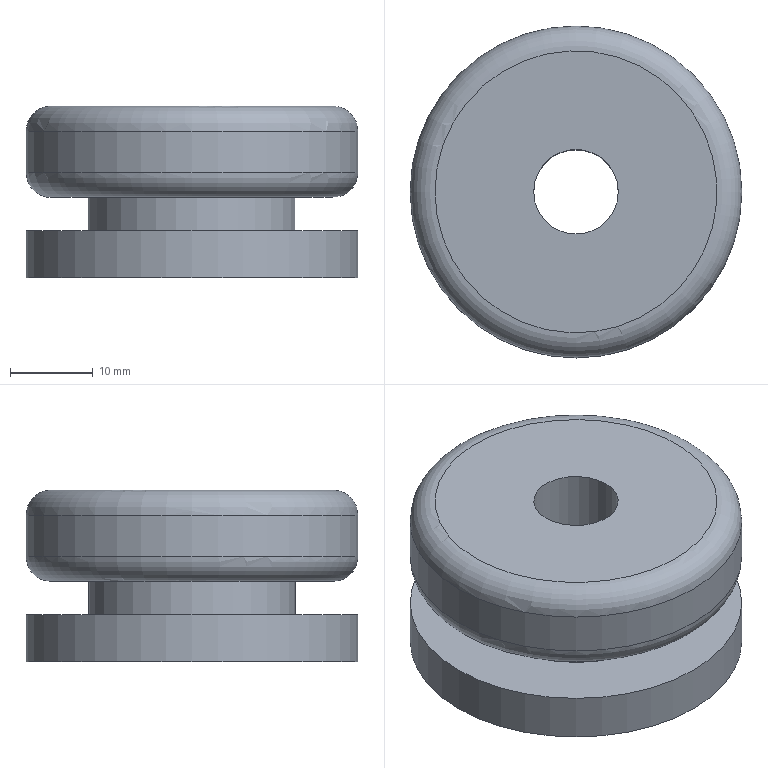Component | NX | RUBBER_PAD_3 | 1 solid | 10 faces | box 40 x 40 x 20.7 mm | volume 20789 mm3 | cylinder 4 | plane 4 | torus 2 | commonest cylinder face diameters 40 x2 10.2 x1 25 x1
STEP:
#1=CARTESIAN_POINT('',(0.,0.,0.));
#2=DIRECTION('',(0.,0.,1.));
#3=DIRECTION('',(1.,0.,0.));
#4=AXIS2_PLACEMENT_3D('',#1,#2,#3);
#5=CARTESIAN_POINT('',(-360.,342.5,-159.7));
#6=VERTEX_POINT('',#5);
#7=CARTESIAN_POINT('',(-340.,342.5,-159.7));
#8=DIRECTION('',(0.,0.,-1.));
#9=DIRECTION('',(-1.,0.,0.));
#10=AXIS2_PLACEMENT_3D('',#7,#8,#9);
#11=CIRCLE('',#10,20.);
#12=CARTESIAN_POINT('',(-340.,342.5,-150.));
#13=DIRECTION('',(0.,0.,-1.));
#14=DIRECTION('',(-1.,0.,0.));
#15=AXIS2_PLACEMENT_3D('',#12,#13,#14);
#16=CYLINDRICAL_SURFACE('',#15,20.);
#17=CARTESIAN_POINT('',(0.,9.7));
#18=DIRECTION('',(1.,0.));
#19=VECTOR('',#18,1.);
#20=LINE('',#17,#19);
#21=(GEOMETRIC_REPRESENTATION_CONTEXT(2)PARAMETRIC_REPRESENTATION_CONTEXT()REPRESENTATION_CONTEXT('',''));
#22=DEFINITIONAL_REPRESENTATION('',(#20),#21);
#23=PCURVE('',#16,#22);
#24=CARTESIAN_POINT('',(-340.,322.5,-159.7));
#25=DIRECTION('',(0.,0.,1.));
#26=DIRECTION('',(1.,0.,0.));
#27=AXIS2_PLACEMENT_3D('',#24,#25,#26);
#28=PLANE('',#27);
#29=CARTESIAN_POINT('',(-20.,20.));
#30=CARTESIAN_POINT('',(-20.,54.641));
#31=CARTESIAN_POINT('',(10.,37.321));
#32=CARTESIAN_POINT('',(40.,20.));
#33=CARTESIAN_POINT('',(10.,2.679));
#34=CARTESIAN_POINT('',(-20.,-14.641));
#35=CARTESIAN_POINT('',(-20.,20.));
#36=(BOUNDED_CURVE()B_SPLINE_CURVE(2,(#29,#30,#31,#32,#33,#34,#35),.UNSPECIFIED.,.T.,.F.)B_SPLINE_CURVE_WITH_KNOTS((1,2,2,2,2,1),(-2.094,0.,2.094,4.189,6.283,8.378),.UNSPECIFIED.)CURVE()GEOMETRIC_REPRESENTATION_ITEM()RATIONAL_B_SPLINE_CURVE((1.,0.5,1.,0.5,1.,0.5,1.))REPRESENTATION_ITEM(''));
#37=(GEOMETRIC_REPRESENTATION_CONTEXT(2)PARAMETRIC_REPRESENTATION_CONTEXT()REPRESENTATION_CONTEXT('',''));
#38=DEFINITIONAL_REPRESENTATION('',(#36),#37);
#39=PCURVE('',#28,#38);
#40=SURFACE_CURVE('',#11,(#23,#39),.PCURVE_S1.);
#41=EDGE_CURVE('',#6,#6,#40,.T.);
#42=ORIENTED_EDGE('',*,*,#41,.F.);
#43=CARTESIAN_POINT('',(-360.,342.5,-154.));
#44=VERTEX_POINT('',#43);
#45=CARTESIAN_POINT('',(-360.,342.5,-154.));
#46=CARTESIAN_POINT('',(-360.,342.5,-159.7));
#47=B_SPLINE_CURVE_WITH_KNOTS('',1,(#45,#46),.UNSPECIFIED.,.F.,.F.,(2,2),(4.,9.7),.PIECEWISE_BEZIER_KNOTS.);
#48=CARTESIAN_POINT('',(0.,0.));
#49=DIRECTION('',(0.,1.));
#50=VECTOR('',#49,1.);
#51=LINE('',#48,#50);
#52=(GEOMETRIC_REPRESENTATION_CONTEXT(2)PARAMETRIC_REPRESENTATION_CONTEXT()REPRESENTATION_CONTEXT('',''));
#53=DEFINITIONAL_REPRESENTATION('',(#51),#52);
#54=PCURVE('',#16,#53);
#55=CARTESIAN_POINT('',(6.283,0.));
#56=DIRECTION('',(0.,1.));
#57=VECTOR('',#56,1.);
#58=LINE('',#55,#57);
#59=(GEOMETRIC_REPRESENTATION_CONTEXT(2)PARAMETRIC_REPRESENTATION_CONTEXT()REPRESENTATION_CONTEXT('',''));
#60=DEFINITIONAL_REPRESENTATION('',(#58),#59);
#61=PCURVE('',#16,#60);
#62=SEAM_CURVE('',#47,(#54,#61),.PCURVE_S1.);
#63=EDGE_CURVE('',#44,#6,#62,.T.);
#64=ORIENTED_EDGE('',*,*,#63,.F.);
#65=CARTESIAN_POINT('',(-340.,342.5,-154.));
#66=DIRECTION('',(0.,0.,-1.));
#67=DIRECTION('',(-1.,0.,0.));
#68=AXIS2_PLACEMENT_3D('',#65,#66,#67);
#69=CIRCLE('',#68,20.);
#70=CARTESIAN_POINT('',(0.,4.));
#71=DIRECTION('',(1.,0.));
#72=VECTOR('',#71,1.);
#73=LINE('',#70,#72);
#74=(GEOMETRIC_REPRESENTATION_CONTEXT(2)PARAMETRIC_REPRESENTATION_CONTEXT()REPRESENTATION_CONTEXT('',''));
#75=DEFINITIONAL_REPRESENTATION('',(#73),#74);
#76=PCURVE('',#16,#75);
#77=CARTESIAN_POINT('',(-340.,330.,-154.));
#78=DIRECTION('',(0.,0.,-1.));
#79=DIRECTION('',(-1.,0.,0.));
#80=AXIS2_PLACEMENT_3D('',#77,#78,#79);
#81=PLANE('',#80);
#82=CARTESIAN_POINT('',(0.,12.5));
#83=DIRECTION('',(1.,0.));
#84=AXIS2_PLACEMENT_2D('',#82,#83);
#85=CIRCLE('',#84,20.);
#86=(GEOMETRIC_REPRESENTATION_CONTEXT(2)PARAMETRIC_REPRESENTATION_CONTEXT()REPRESENTATION_CONTEXT('',''));
#87=DEFINITIONAL_REPRESENTATION('',(#85),#86);
#88=PCURVE('',#81,#87);
#89=SURFACE_CURVE('',#69,(#76,#88),.PCURVE_S1.);
#90=EDGE_CURVE('',#44,#44,#89,.T.);
#91=ORIENTED_EDGE('',*,*,#90,.T.);
#92=ORIENTED_EDGE('',*,*,#63,.T.);
#93=EDGE_LOOP('',(#42,#64,#91,#92));
#94=FACE_BOUND('',#93,.T.);
#95=ADVANCED_FACE('',(#94),#16,.T.);
#96=CARTESIAN_POINT('',(-345.1,342.5,-159.7));
#97=VERTEX_POINT('',#96);
#98=CARTESIAN_POINT('',(-340.,342.5,-159.7));
#99=DIRECTION('',(0.,0.,-1.));
#100=DIRECTION('',(-1.,0.,0.));
#101=AXIS2_PLACEMENT_3D('',#98,#99,#100);
#102=CIRCLE('',#101,5.1);
#103=CARTESIAN_POINT('',(-5.1,20.));
#104=CARTESIAN_POINT('',(-5.1,28.833));
#105=CARTESIAN_POINT('',(2.55,24.417));
#106=CARTESIAN_POINT('',(10.2,20.));
#107=CARTESIAN_POINT('',(2.55,15.583));
#108=CARTESIAN_POINT('',(-5.1,11.167));
#109=CARTESIAN_POINT('',(-5.1,20.));
#110=(BOUNDED_CURVE()B_SPLINE_CURVE(2,(#103,#104,#105,#106,#107,#108,#109),.UNSPECIFIED.,.T.,.F.)B_SPLINE_CURVE_WITH_KNOTS((1,2,2,2,2,1),(-2.094,0.,2.094,4.189,6.283,8.378),.UNSPECIFIED.)CURVE()GEOMETRIC_REPRESENTATION_ITEM()RATIONAL_B_SPLINE_CURVE((1.,0.5,1.,0.5,1.,0.5,1.))REPRESENTATION_ITEM(''));
#111=(GEOMETRIC_REPRESENTATION_CONTEXT(2)PARAMETRIC_REPRESENTATION_CONTEXT()REPRESENTATION_CONTEXT('',''));
#112=DEFINITIONAL_REPRESENTATION('',(#110),#111);
#113=PCURVE('',#28,#112);
#114=CARTESIAN_POINT('',(-340.,342.5,-150.));
#115=DIRECTION('',(0.,0.,-1.));
#116=DIRECTION('',(-1.,0.,0.));
#117=AXIS2_PLACEMENT_3D('',#114,#115,#116);
#118=CYLINDRICAL_SURFACE('',#117,5.1);
#119=CARTESIAN_POINT('',(0.,9.7));
#120=DIRECTION('',(1.,0.));
#121=VECTOR('',#120,1.);
#122=LINE('',#119,#121);
#123=(GEOMETRIC_REPRESENTATION_CONTEXT(2)PARAMETRIC_REPRESENTATION_CONTEXT()REPRESENTATION_CONTEXT('',''));
#124=DEFINITIONAL_REPRESENTATION('',(#122),#123);
#125=PCURVE('',#118,#124);
#126=SURFACE_CURVE('',#102,(#113,#125),.PCURVE_S1.);
#127=EDGE_CURVE('',#97,#97,#126,.T.);
#128=ORIENTED_EDGE('',*,*,#127,.F.);
#129=EDGE_LOOP('',(#128));
#130=FACE_BOUND('',#129,.T.);
#131=ORIENTED_EDGE('',*,*,#41,.T.);
#132=EDGE_LOOP('',(#131));
#133=FACE_BOUND('',#132,.T.);
#134=ADVANCED_FACE('',(#130,#133),#28,.F.);
#135=CARTESIAN_POINT('',(-345.1,342.5,-139.));
#136=VERTEX_POINT('',#135);
#137=CARTESIAN_POINT('',(-340.,342.5,-139.));
#138=DIRECTION('',(0.,0.,-1.));
#139=DIRECTION('',(-1.,0.,0.));
#140=AXIS2_PLACEMENT_3D('',#137,#138,#139);
#141=CIRCLE('',#140,5.1);
#142=CARTESIAN_POINT('',(0.,-11.));
#143=DIRECTION('',(1.,0.));
#144=VECTOR('',#143,1.);
#145=LINE('',#142,#144);
#146=(GEOMETRIC_REPRESENTATION_CONTEXT(2)PARAMETRIC_REPRESENTATION_CONTEXT()REPRESENTATION_CONTEXT('',''));
#147=DEFINITIONAL_REPRESENTATION('',(#145),#146);
#148=PCURVE('',#118,#147);
#149=CARTESIAN_POINT('',(-340.,337.4,-139.));
#150=DIRECTION('',(0.,0.,-1.));
#151=DIRECTION('',(-1.,0.,0.));
#152=AXIS2_PLACEMENT_3D('',#149,#150,#151);
#153=PLANE('',#152);
#154=CARTESIAN_POINT('',(0.,5.1));
#155=DIRECTION('',(1.,0.));
#156=AXIS2_PLACEMENT_2D('',#154,#155);
#157=CIRCLE('',#156,5.1);
#158=(GEOMETRIC_REPRESENTATION_CONTEXT(2)PARAMETRIC_REPRESENTATION_CONTEXT()REPRESENTATION_CONTEXT('',''));
#159=DEFINITIONAL_REPRESENTATION('',(#157),#158);
#160=PCURVE('',#153,#159);
#161=SURFACE_CURVE('',#141,(#148,#160),.PCURVE_S1.);
#162=EDGE_CURVE('',#136,#136,#161,.T.);
#163=ORIENTED_EDGE('',*,*,#162,.T.);
#164=CARTESIAN_POINT('',(-345.1,342.5,-139.));
#165=CARTESIAN_POINT('',(-345.1,342.5,-159.7));
#166=B_SPLINE_CURVE_WITH_KNOTS('',1,(#164,#165),.UNSPECIFIED.,.F.,.F.,(2,2),(-11.,9.7),.PIECEWISE_BEZIER_KNOTS.);
#167=CARTESIAN_POINT('',(6.283,0.));
#168=DIRECTION('',(0.,1.));
#169=VECTOR('',#168,1.);
#170=LINE('',#167,#169);
#171=(GEOMETRIC_REPRESENTATION_CONTEXT(2)PARAMETRIC_REPRESENTATION_CONTEXT()REPRESENTATION_CONTEXT('',''));
#172=DEFINITIONAL_REPRESENTATION('',(#170),#171);
#173=PCURVE('',#118,#172);
#174=CARTESIAN_POINT('',(0.,0.));
#175=DIRECTION('',(0.,1.));
#176=VECTOR('',#175,1.);
#177=LINE('',#174,#176);
#178=(GEOMETRIC_REPRESENTATION_CONTEXT(2)PARAMETRIC_REPRESENTATION_CONTEXT()REPRESENTATION_CONTEXT('',''));
#179=DEFINITIONAL_REPRESENTATION('',(#177),#178);
#180=PCURVE('',#118,#179);
#181=SEAM_CURVE('',#166,(#173,#180),.PCURVE_S1.);
#182=EDGE_CURVE('',#136,#97,#181,.T.);
#183=ORIENTED_EDGE('',*,*,#182,.T.);
#184=ORIENTED_EDGE('',*,*,#127,.F.);
#185=ORIENTED_EDGE('',*,*,#182,.F.);
#186=EDGE_LOOP('',(#163,#183,#184,#185));
#187=FACE_BOUND('',#186,.F.);
#188=ADVANCED_FACE('',(#187),#118,.F.);
#189=CARTESIAN_POINT('',(-357.,342.5,-139.));
#190=VERTEX_POINT('',#189);
#191=CARTESIAN_POINT('',(-340.,342.5,-139.));
#192=DIRECTION('',(0.,0.,-1.));
#193=DIRECTION('',(-1.,0.,0.));
#194=AXIS2_PLACEMENT_3D('',#191,#192,#193);
#195=CIRCLE('',#194,17.);
#196=CARTESIAN_POINT('',(0.,5.1));
#197=DIRECTION('',(1.,0.));
#198=AXIS2_PLACEMENT_2D('',#196,#197);
#199=CIRCLE('',#198,17.);
#200=(GEOMETRIC_REPRESENTATION_CONTEXT(2)PARAMETRIC_REPRESENTATION_CONTEXT()REPRESENTATION_CONTEXT('',''));
#201=DEFINITIONAL_REPRESENTATION('',(#199),#200);
#202=PCURVE('',#153,#201);
#203=CARTESIAN_POINT('',(-340.,342.5,-142.));
#204=DIRECTION('',(0.,0.,-1.));
#205=DIRECTION('',(-1.,0.,0.));
#206=AXIS2_PLACEMENT_3D('',#203,#204,#205);
#207=TOROIDAL_SURFACE('',#206,17.,3.);
#208=CARTESIAN_POINT('',(0.,4.712));
#209=DIRECTION('',(1.,0.));
#210=VECTOR('',#209,1.);
#211=LINE('',#208,#210);
#212=(GEOMETRIC_REPRESENTATION_CONTEXT(2)PARAMETRIC_REPRESENTATION_CONTEXT()REPRESENTATION_CONTEXT('',''));
#213=DEFINITIONAL_REPRESENTATION('',(#211),#212);
#214=PCURVE('',#207,#213);
#215=SURFACE_CURVE('',#195,(#202,#214),.PCURVE_S1.);
#216=EDGE_CURVE('',#190,#190,#215,.T.);
#217=ORIENTED_EDGE('',*,*,#216,.F.);
#218=EDGE_LOOP('',(#217));
#219=FACE_BOUND('',#218,.T.);
#220=ORIENTED_EDGE('',*,*,#162,.T.);
#221=EDGE_LOOP('',(#220));
#222=FACE_BOUND('',#221,.T.);
#223=ADVANCED_FACE('',(#219,#222),#153,.F.);
#224=CARTESIAN_POINT('',(-360.,342.5,-142.));
#225=VERTEX_POINT('',#224);
#226=CARTESIAN_POINT('',(-340.,342.5,-142.));
#227=DIRECTION('',(0.,0.,-1.));
#228=DIRECTION('',(-1.,0.,0.));
#229=AXIS2_PLACEMENT_3D('',#226,#227,#228);
#230=CIRCLE('',#229,20.);
#231=CARTESIAN_POINT('',(0.,6.283));
#232=DIRECTION('',(1.,0.));
#233=VECTOR('',#232,1.);
#234=LINE('',#231,#233);
#235=(GEOMETRIC_REPRESENTATION_CONTEXT(2)PARAMETRIC_REPRESENTATION_CONTEXT()REPRESENTATION_CONTEXT('',''));
#236=DEFINITIONAL_REPRESENTATION('',(#234),#235);
#237=PCURVE('',#207,#236);
#238=CARTESIAN_POINT('',(-340.,342.5,-150.));
#239=DIRECTION('',(0.,0.,-1.));
#240=DIRECTION('',(-1.,0.,0.));
#241=AXIS2_PLACEMENT_3D('',#238,#239,#240);
#242=CYLINDRICAL_SURFACE('',#241,20.);
#243=CARTESIAN_POINT('',(0.,-8.));
#244=DIRECTION('',(1.,0.));
#245=VECTOR('',#244,1.);
#246=LINE('',#243,#245);
#247=(GEOMETRIC_REPRESENTATION_CONTEXT(2)PARAMETRIC_REPRESENTATION_CONTEXT()REPRESENTATION_CONTEXT('',''));
#248=DEFINITIONAL_REPRESENTATION('',(#246),#247);
#249=PCURVE('',#242,#248);
#250=SURFACE_CURVE('',#230,(#237,#249),.PCURVE_S1.);
#251=EDGE_CURVE('',#225,#225,#250,.T.);
#252=ORIENTED_EDGE('',*,*,#251,.F.);
#253=CARTESIAN_POINT('',(-357.,342.5,-139.));
#254=CARTESIAN_POINT('',(-357.802,342.5,-139.));
#255=CARTESIAN_POINT('',(-358.583,342.5,-139.255));
#256=CARTESIAN_POINT('',(-359.256,342.5,-139.744));
#257=CARTESIAN_POINT('',(-359.745,342.5,-140.417));
#258=CARTESIAN_POINT('',(-360.,342.5,-141.198));
#259=CARTESIAN_POINT('',(-360.,342.5,-142.));
#260=(BOUNDED_CURVE()B_SPLINE_CURVE(6,(#253,#254,#255,#256,#257,#258,#259),.UNSPECIFIED.,.F.,.F.)B_SPLINE_CURVE_WITH_KNOTS((7,7),(-1.571,0.),.PIECEWISE_BEZIER_KNOTS.)CURVE()GEOMETRIC_REPRESENTATION_ITEM()RATIONAL_B_SPLINE_CURVE((1.031,1.01,0.9979,0.994,0.9979,1.01,1.031))REPRESENTATION_ITEM(''));
#261=CARTESIAN_POINT('',(0.,6.283));
#262=DIRECTION('',(0.,1.));
#263=VECTOR('',#262,1.);
#264=LINE('',#261,#263);
#265=(GEOMETRIC_REPRESENTATION_CONTEXT(2)PARAMETRIC_REPRESENTATION_CONTEXT()REPRESENTATION_CONTEXT('',''));
#266=DEFINITIONAL_REPRESENTATION('',(#264),#265);
#267=PCURVE('',#207,#266);
#268=CARTESIAN_POINT('',(6.283,6.283));
#269=DIRECTION('',(0.,1.));
#270=VECTOR('',#269,1.);
#271=LINE('',#268,#270);
#272=(GEOMETRIC_REPRESENTATION_CONTEXT(2)PARAMETRIC_REPRESENTATION_CONTEXT()REPRESENTATION_CONTEXT('',''));
#273=DEFINITIONAL_REPRESENTATION('',(#271),#272);
#274=PCURVE('',#207,#273);
#275=SEAM_CURVE('',#260,(#267,#274),.PCURVE_S1.);
#276=EDGE_CURVE('',#190,#225,#275,.T.);
#277=ORIENTED_EDGE('',*,*,#276,.F.);
#278=ORIENTED_EDGE('',*,*,#216,.T.);
#279=ORIENTED_EDGE('',*,*,#276,.T.);
#280=EDGE_LOOP('',(#252,#277,#278,#279));
#281=FACE_BOUND('',#280,.T.);
#282=ADVANCED_FACE('',(#281),#207,.T.);
#283=CARTESIAN_POINT('',(-360.,342.5,-147.));
#284=VERTEX_POINT('',#283);
#285=CARTESIAN_POINT('',(-340.,342.5,-147.));
#286=DIRECTION('',(0.,0.,-1.));
#287=DIRECTION('',(-1.,0.,0.));
#288=AXIS2_PLACEMENT_3D('',#285,#286,#287);
#289=CIRCLE('',#288,20.);
#290=CARTESIAN_POINT('',(0.,-3.));
#291=DIRECTION('',(1.,0.));
#292=VECTOR('',#291,1.);
#293=LINE('',#290,#292);
#294=(GEOMETRIC_REPRESENTATION_CONTEXT(2)PARAMETRIC_REPRESENTATION_CONTEXT()REPRESENTATION_CONTEXT('',''));
#295=DEFINITIONAL_REPRESENTATION('',(#293),#294);
#296=PCURVE('',#242,#295);
#297=CARTESIAN_POINT('',(-340.,342.5,-147.));
#298=DIRECTION('',(0.,0.,-1.));
#299=DIRECTION('',(-1.,0.,0.));
#300=AXIS2_PLACEMENT_3D('',#297,#298,#299);
#301=TOROIDAL_SURFACE('',#300,17.,3.);
#302=CARTESIAN_POINT('',(0.,6.283));
#303=DIRECTION('',(1.,0.));
#304=VECTOR('',#303,1.);
#305=LINE('',#302,#304);
#306=(GEOMETRIC_REPRESENTATION_CONTEXT(2)PARAMETRIC_REPRESENTATION_CONTEXT()REPRESENTATION_CONTEXT('',''));
#307=DEFINITIONAL_REPRESENTATION('',(#305),#306);
#308=PCURVE('',#301,#307);
#309=SURFACE_CURVE('',#289,(#296,#308),.PCURVE_S1.);
#310=EDGE_CURVE('',#284,#284,#309,.T.);
#311=ORIENTED_EDGE('',*,*,#310,.F.);
#312=CARTESIAN_POINT('',(-360.,342.5,-142.));
#313=CARTESIAN_POINT('',(-360.,342.5,-147.));
#314=B_SPLINE_CURVE_WITH_KNOTS('',1,(#312,#313),.UNSPECIFIED.,.F.,.F.,(2,2),(-8.,-3.),.PIECEWISE_BEZIER_KNOTS.);
#315=CARTESIAN_POINT('',(0.,0.));
#316=DIRECTION('',(0.,1.));
#317=VECTOR('',#316,1.);
#318=LINE('',#315,#317);
#319=(GEOMETRIC_REPRESENTATION_CONTEXT(2)PARAMETRIC_REPRESENTATION_CONTEXT()REPRESENTATION_CONTEXT('',''));
#320=DEFINITIONAL_REPRESENTATION('',(#318),#319);
#321=PCURVE('',#242,#320);
#322=CARTESIAN_POINT('',(6.283,0.));
#323=DIRECTION('',(0.,1.));
#324=VECTOR('',#323,1.);
#325=LINE('',#322,#324);
#326=(GEOMETRIC_REPRESENTATION_CONTEXT(2)PARAMETRIC_REPRESENTATION_CONTEXT()REPRESENTATION_CONTEXT('',''));
#327=DEFINITIONAL_REPRESENTATION('',(#325),#326);
#328=PCURVE('',#242,#327);
#329=SEAM_CURVE('',#314,(#321,#328),.PCURVE_S1.);
#330=EDGE_CURVE('',#225,#284,#329,.T.);
#331=ORIENTED_EDGE('',*,*,#330,.F.);
#332=ORIENTED_EDGE('',*,*,#251,.T.);
#333=ORIENTED_EDGE('',*,*,#330,.T.);
#334=EDGE_LOOP('',(#311,#331,#332,#333));
#335=FACE_BOUND('',#334,.T.);
#336=ADVANCED_FACE('',(#335),#242,.T.);
#337=CARTESIAN_POINT('',(-357.,342.5,-150.));
#338=VERTEX_POINT('',#337);
#339=CARTESIAN_POINT('',(-340.,342.5,-150.));
#340=DIRECTION('',(0.,0.,-1.));
#341=DIRECTION('',(-1.,0.,0.));
#342=AXIS2_PLACEMENT_3D('',#339,#340,#341);
#343=CIRCLE('',#342,17.);
#344=CARTESIAN_POINT('',(0.,7.854));
#345=DIRECTION('',(1.,0.));
#346=VECTOR('',#345,1.);
#347=LINE('',#344,#346);
#348=(GEOMETRIC_REPRESENTATION_CONTEXT(2)PARAMETRIC_REPRESENTATION_CONTEXT()REPRESENTATION_CONTEXT('',''));
#349=DEFINITIONAL_REPRESENTATION('',(#347),#348);
#350=PCURVE('',#301,#349);
#351=CARTESIAN_POINT('',(-340.,325.5,-150.));
#352=DIRECTION('',(0.,0.,1.));
#353=DIRECTION('',(1.,0.,0.));
#354=AXIS2_PLACEMENT_3D('',#351,#352,#353);
#355=PLANE('',#354);
#356=CARTESIAN_POINT('',(-17.,17.));
#357=CARTESIAN_POINT('',(-17.,46.445));
#358=CARTESIAN_POINT('',(8.5,31.722));
#359=CARTESIAN_POINT('',(34.,17.));
#360=CARTESIAN_POINT('',(8.5,2.278));
#361=CARTESIAN_POINT('',(-17.,-12.445));
#362=CARTESIAN_POINT('',(-17.,17.));
#363=(BOUNDED_CURVE()B_SPLINE_CURVE(2,(#356,#357,#358,#359,#360,#361,#362),.UNSPECIFIED.,.T.,.F.)B_SPLINE_CURVE_WITH_KNOTS((1,2,2,2,2,1),(-2.094,0.,2.094,4.189,6.283,8.378),.UNSPECIFIED.)CURVE()GEOMETRIC_REPRESENTATION_ITEM()RATIONAL_B_SPLINE_CURVE((1.,0.5,1.,0.5,1.,0.5,1.))REPRESENTATION_ITEM(''));
#364=(GEOMETRIC_REPRESENTATION_CONTEXT(2)PARAMETRIC_REPRESENTATION_CONTEXT()REPRESENTATION_CONTEXT('',''));
#365=DEFINITIONAL_REPRESENTATION('',(#363),#364);
#366=PCURVE('',#355,#365);
#367=SURFACE_CURVE('',#343,(#350,#366),.PCURVE_S1.);
#368=EDGE_CURVE('',#338,#338,#367,.T.);
#369=ORIENTED_EDGE('',*,*,#368,.F.);
#370=CARTESIAN_POINT('',(-360.,342.5,-147.));
#371=CARTESIAN_POINT('',(-360.,342.5,-147.802));
#372=CARTESIAN_POINT('',(-359.745,342.5,-148.583));
#373=CARTESIAN_POINT('',(-359.256,342.5,-149.256));
#374=CARTESIAN_POINT('',(-358.583,342.5,-149.745));
#375=CARTESIAN_POINT('',(-357.802,342.5,-150.));
#376=CARTESIAN_POINT('',(-357.,342.5,-150.));
#377=(BOUNDED_CURVE()B_SPLINE_CURVE(6,(#370,#371,#372,#373,#374,#375,#376),.UNSPECIFIED.,.F.,.F.)B_SPLINE_CURVE_WITH_KNOTS((7,7),(0.,1.571),.PIECEWISE_BEZIER_KNOTS.)CURVE()GEOMETRIC_REPRESENTATION_ITEM()RATIONAL_B_SPLINE_CURVE((1.031,1.01,0.9979,0.994,0.9979,1.01,1.031))REPRESENTATION_ITEM(''));
#378=CARTESIAN_POINT('',(0.,6.283));
#379=DIRECTION('',(0.,1.));
#380=VECTOR('',#379,1.);
#381=LINE('',#378,#380);
#382=(GEOMETRIC_REPRESENTATION_CONTEXT(2)PARAMETRIC_REPRESENTATION_CONTEXT()REPRESENTATION_CONTEXT('',''));
#383=DEFINITIONAL_REPRESENTATION('',(#381),#382);
#384=PCURVE('',#301,#383);
#385=CARTESIAN_POINT('',(6.283,6.283));
#386=DIRECTION('',(0.,1.));
#387=VECTOR('',#386,1.);
#388=LINE('',#385,#387);
#389=(GEOMETRIC_REPRESENTATION_CONTEXT(2)PARAMETRIC_REPRESENTATION_CONTEXT()REPRESENTATION_CONTEXT('',''));
#390=DEFINITIONAL_REPRESENTATION('',(#388),#389);
#391=PCURVE('',#301,#390);
#392=SEAM_CURVE('',#377,(#384,#391),.PCURVE_S1.);
#393=EDGE_CURVE('',#284,#338,#392,.T.);
#394=ORIENTED_EDGE('',*,*,#393,.F.);
#395=ORIENTED_EDGE('',*,*,#310,.T.);
#396=ORIENTED_EDGE('',*,*,#393,.T.);
#397=EDGE_LOOP('',(#369,#394,#395,#396));
#398=FACE_BOUND('',#397,.T.);
#399=ADVANCED_FACE('',(#398),#301,.T.);
#400=CARTESIAN_POINT('',(-352.5,342.5,-150.));
#401=VERTEX_POINT('',#400);
#402=CARTESIAN_POINT('',(-340.,342.5,-150.));
#403=DIRECTION('',(0.,0.,-1.));
#404=DIRECTION('',(-1.,0.,0.));
#405=AXIS2_PLACEMENT_3D('',#402,#403,#404);
#406=CIRCLE('',#405,12.5);
#407=CARTESIAN_POINT('',(-12.5,17.));
#408=CARTESIAN_POINT('',(-12.5,38.651));
#409=CARTESIAN_POINT('',(6.25,27.825));
#410=CARTESIAN_POINT('',(25.,17.));
#411=CARTESIAN_POINT('',(6.25,6.175));
#412=CARTESIAN_POINT('',(-12.5,-4.651));
#413=CARTESIAN_POINT('',(-12.5,17.));
#414=(BOUNDED_CURVE()B_SPLINE_CURVE(2,(#407,#408,#409,#410,#411,#412,#413),.UNSPECIFIED.,.T.,.F.)B_SPLINE_CURVE_WITH_KNOTS((1,2,2,2,2,1),(-2.094,0.,2.094,4.189,6.283,8.378),.UNSPECIFIED.)CURVE()GEOMETRIC_REPRESENTATION_ITEM()RATIONAL_B_SPLINE_CURVE((1.,0.5,1.,0.5,1.,0.5,1.))REPRESENTATION_ITEM(''));
#415=(GEOMETRIC_REPRESENTATION_CONTEXT(2)PARAMETRIC_REPRESENTATION_CONTEXT()REPRESENTATION_CONTEXT('',''));
#416=DEFINITIONAL_REPRESENTATION('',(#414),#415);
#417=PCURVE('',#355,#416);
#418=CARTESIAN_POINT('',(-340.,342.5,-150.));
#419=DIRECTION('',(0.,0.,-1.));
#420=DIRECTION('',(-1.,0.,0.));
#421=AXIS2_PLACEMENT_3D('',#418,#419,#420);
#422=CYLINDRICAL_SURFACE('',#421,12.5);
#423=CARTESIAN_POINT('',(0.,0.));
#424=DIRECTION('',(1.,0.));
#425=VECTOR('',#424,1.);
#426=LINE('',#423,#425);
#427=(GEOMETRIC_REPRESENTATION_CONTEXT(2)PARAMETRIC_REPRESENTATION_CONTEXT()REPRESENTATION_CONTEXT('',''));
#428=DEFINITIONAL_REPRESENTATION('',(#426),#427);
#429=PCURVE('',#422,#428);
#430=SURFACE_CURVE('',#406,(#417,#429),.PCURVE_S1.);
#431=EDGE_CURVE('',#401,#401,#430,.T.);
#432=ORIENTED_EDGE('',*,*,#431,.F.);
#433=EDGE_LOOP('',(#432));
#434=FACE_BOUND('',#433,.T.);
#435=ORIENTED_EDGE('',*,*,#368,.T.);
#436=EDGE_LOOP('',(#435));
#437=FACE_BOUND('',#436,.T.);
#438=ADVANCED_FACE('',(#434,#437),#355,.F.);
#439=CARTESIAN_POINT('',(-352.5,342.5,-154.));
#440=VERTEX_POINT('',#439);
#441=CARTESIAN_POINT('',(-340.,342.5,-154.));
#442=DIRECTION('',(0.,0.,-1.));
#443=DIRECTION('',(-1.,0.,0.));
#444=AXIS2_PLACEMENT_3D('',#441,#442,#443);
#445=CIRCLE('',#444,12.5);
#446=CARTESIAN_POINT('',(0.,4.));
#447=DIRECTION('',(1.,0.));
#448=VECTOR('',#447,1.);
#449=LINE('',#446,#448);
#450=(GEOMETRIC_REPRESENTATION_CONTEXT(2)PARAMETRIC_REPRESENTATION_CONTEXT()REPRESENTATION_CONTEXT('',''));
#451=DEFINITIONAL_REPRESENTATION('',(#449),#450);
#452=PCURVE('',#422,#451);
#453=CARTESIAN_POINT('',(0.,12.5));
#454=DIRECTION('',(1.,0.));
#455=AXIS2_PLACEMENT_2D('',#453,#454);
#456=CIRCLE('',#455,12.5);
#457=(GEOMETRIC_REPRESENTATION_CONTEXT(2)PARAMETRIC_REPRESENTATION_CONTEXT()REPRESENTATION_CONTEXT('',''));
#458=DEFINITIONAL_REPRESENTATION('',(#456),#457);
#459=PCURVE('',#81,#458);
#460=SURFACE_CURVE('',#445,(#452,#459),.PCURVE_S1.);
#461=EDGE_CURVE('',#440,#440,#460,.T.);
#462=ORIENTED_EDGE('',*,*,#461,.F.);
#463=CARTESIAN_POINT('',(-352.5,342.5,-150.));
#464=CARTESIAN_POINT('',(-352.5,342.5,-154.));
#465=B_SPLINE_CURVE_WITH_KNOTS('',1,(#463,#464),.UNSPECIFIED.,.F.,.F.,(2,2),(0.,4.),.PIECEWISE_BEZIER_KNOTS.);
#466=CARTESIAN_POINT('',(0.,0.));
#467=DIRECTION('',(0.,1.));
#468=VECTOR('',#467,1.);
#469=LINE('',#466,#468);
#470=(GEOMETRIC_REPRESENTATION_CONTEXT(2)PARAMETRIC_REPRESENTATION_CONTEXT()REPRESENTATION_CONTEXT('',''));
#471=DEFINITIONAL_REPRESENTATION('',(#469),#470);
#472=PCURVE('',#422,#471);
#473=CARTESIAN_POINT('',(6.283,0.));
#474=DIRECTION('',(0.,1.));
#475=VECTOR('',#474,1.);
#476=LINE('',#473,#475);
#477=(GEOMETRIC_REPRESENTATION_CONTEXT(2)PARAMETRIC_REPRESENTATION_CONTEXT()REPRESENTATION_CONTEXT('',''));
#478=DEFINITIONAL_REPRESENTATION('',(#476),#477);
#479=PCURVE('',#422,#478);
#480=SEAM_CURVE('',#465,(#472,#479),.PCURVE_S1.);
#481=EDGE_CURVE('',#401,#440,#480,.T.);
#482=ORIENTED_EDGE('',*,*,#481,.F.);
#483=ORIENTED_EDGE('',*,*,#431,.T.);
#484=ORIENTED_EDGE('',*,*,#481,.T.);
#485=EDGE_LOOP('',(#462,#482,#483,#484));
#486=FACE_BOUND('',#485,.T.);
#487=ADVANCED_FACE('',(#486),#422,.T.);
#488=ORIENTED_EDGE('',*,*,#90,.F.);
#489=EDGE_LOOP('',(#488));
#490=FACE_BOUND('',#489,.T.);
#491=ORIENTED_EDGE('',*,*,#461,.T.);
#492=EDGE_LOOP('',(#491));
#493=FACE_BOUND('',#492,.T.);
#494=ADVANCED_FACE('',(#490,#493),#81,.F.);
#495=CLOSED_SHELL('',(#95,#134,#188,#223,#282,#336,#399,#438,#487,#494));
#496=MANIFOLD_SOLID_BREP('',#495);
#497=(LENGTH_UNIT()NAMED_UNIT(*)SI_UNIT(.MILLI.,.METRE.));
#498=UNCERTAINTY_MEASURE_WITH_UNIT(LENGTH_MEASURE(0.00001),#497,'','');
#499=(NAMED_UNIT(*)PLANE_ANGLE_UNIT()SI_UNIT($,.RADIAN.));
#500=(NAMED_UNIT(*)SI_UNIT($,.STERADIAN.)SOLID_ANGLE_UNIT());
#501=(GEOMETRIC_REPRESENTATION_CONTEXT(3)GLOBAL_UNCERTAINTY_ASSIGNED_CONTEXT((#498))GLOBAL_UNIT_ASSIGNED_CONTEXT((#497,#499,#500))REPRESENTATION_CONTEXT('',''));
#502=ADVANCED_BREP_SHAPE_REPRESENTATION('',(#4,#496),#501);